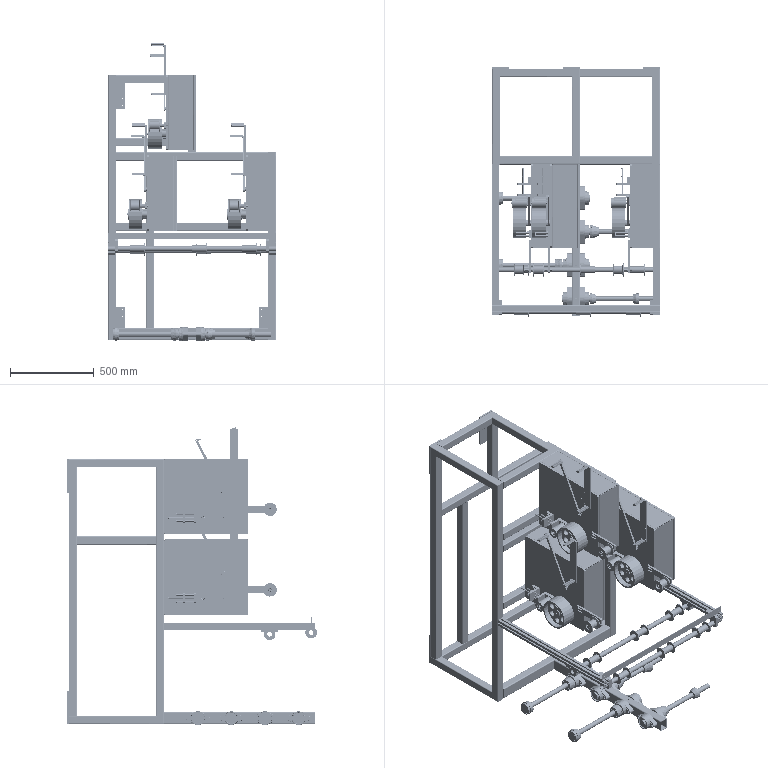Assembly | SolidWorks | mm | 185 component files | 205 solids | 13372 faces | box 1000 x 1490 x 1777.99 mm | volume 37448972 mm3 | plane 5170 | cylinder 3628 | spline 2452 | torus 1200 | sphere 624 | cone 298 | commonest cylinder face diameters 107 x315 102.497 x315 6 x255 5 x252 10 x167 4.2 x152 32.5 x120 36.5 x114
Bill of materials:
291_UCFLU206 | 8 |  | Two-bolt flange housing with a diamond/oval base. It has a raised round boss holding an inner ring with a bore, and a small protrusion on the rim that looks like a nipple.
AluminumBracket | 2 |  | Long straight bar with a square, slotted cross-section that stays the same along its length, made of four corner lobes around a central core.
Axis | 4 |  | Plain solid round rod with flat ends.
AxisSeat | 2 |  | Block with a wide flat top flange and a narrower lower body that has a large horizontal through bore and chamfered lower corners.
BearingBasePlate | 8 |  | Flat diamond-shaped plate or spacer with rounded ends, a large central hole and two small holes at the ends.
AdjustmentSeat | 3 |  | Thick L-shaped angle bracket with slotted holes in both legs and small holes in the end face of the long leg.
AngleDisplacementSensor | 3 |  | Stepped round part: a small shaft stub, a middle step and a large cylindrical head with a narrow ring groove near the shoulder.
AngleDisplacementSensorMountingPlate | 3 |  | Flat plate with two chamfered corners at the bottom, two small holes near the top and one large hole near the bottom.
AngleDisplacementSensorNut | 3 |  | Hexagonal ring shaped like a thin nut, with a large plain round bore.
AngleSensorConnectionAxis | 3 |  | Stepped round shaft with a raised collar, a hollow end with a central bore and two small cross holes near that end.
BearingHousing2 | 3 |  | Near-cubic block with a stepped (counterbored) horizontal through bore, two holes in the top face and one chamfered lower edge.
CylindricalGear35_1 | 3 | 45 | Straight-toothed spur gear with a plain central bore and radial holes through the rim into the bore.
deep groove ball bearings gb | 24 |  | Ring-shaped rolling-element assembly shape: outer ring and inner ring with a single row of spherical balls between them, resembling a radial ball bearing.
AuxiliaryWheel | 3 |  | Cylindrical sleeve with a thin raised flange at each end and a central through bore.
AuxiliaryWheelAdjustmentSeat | 3 |  | L-shaped angle bracket of roughly uniform thickness: one leg has three round holes in a line, the other leg has two parallel elongated slots.
AuxiliaryWheelFrame | 3 |  | L-shaped angle bracket: one leg has three small round holes in a line, the other leg has a single round hole.
BearingHousing | 3 |  | Thick rectangular block or plate with a large central circular through hole and four smaller round holes near the corners.
CopperSleeve10-14 | 9 |  | Plain cylindrical tube or sleeve with a concentric through bore and flat ends.
CylindricalGear105_1 | 3 | 45 | Thin flat disc-type spur gear with many small external teeth and a central bore with a single keyway notch.
ElectricalBoxCover | 3 |  | Thin flat rectangular plate or panel with no clear holes or cutouts.
GuidePlate | 3 |  | Long narrow flat bar or plate with a pattern of small round holes: two pairs of larger holes toward one end and a single smaller hole near each end.
GuidePlate2 | 3 |  | Rectangular flat bar with chamfered corners at one end, a single round hole near that end, and two parallel elongated slots near the opposite end.
GuideWheel | 3 |  | Cylindrical wheel or drum: an outer rim surrounds a recessed web with six round lightening-style holes around a central hub with a keyed bore.
M6-8-13-100GuidePinBolt | 6 |  | Headed stepped cylindrical pin: a short larger-diameter head, a long main shank, and a reduced-diameter tip section at the far end.
M6-8-13-150GuidePinBolt | 3 |  | Long, slender solid round pin. It has a short larger-diameter cylindrical head at one end and a small stepped-down end at the other.
M8-10-16-90GuidePinBolt | 3 |  | Solid round pin with a cylindrical head. The head joins a main shank through a short neck. At the far end the shank steps down through a short collar section to a reduced-diameter tip.
MotorShaftSleeve | 3 |  | Hollow cylindrical sleeve with two outside diameters. It has a keyed through-bore, and the larger-diameter section has small radial cross holes.
MotorShaftSleeve2 | 3 |  | Flanged tubular spacer: a thin circular flange at one end of a cylindrical tube with a small central through-hole.
NylonGuideBlock | 9 |  | Long rectangular-section, U-shaped fork-like bar: two parallel prongs joined at one end, leaving a long open slot between them. One prong ends in a taller block with a transverse round hole.
Part6 | 3 |  | Thin, flat rectangular plate with chamfered corners. It has two larger round holes and a pattern of many small holes.
RollerAxis | 3 |  | Round shaft with a larger cylindrical collar placed off-center along its length. The collar has a flat face on one side, and the shaft continues from both ends of the collar at slightly different diameters.
RoundNut | 3 |  | Short, thick annular ring with a large central bore and several rectangular notches spaced around its outer edge.
SmallElectricalBox | 3 |  | Thin-walled rectangular box or enclosure that is open on one large face. The opposite wall has one large round hole, one smaller round hole, and several small holes.
StepperMotor | 3 |  | Compact block-shaped body with a square end flange that has a mounting hole near each corner. A cylindrical boss projects from one end and a stepped round shaft from the other, and the body's long edges have grooves.
SwingArm | 3 |  | Long, slender rectangular-section bar or strip with a round hole near each end. The two holes appear to be different sizes.
SwingRodAxis | 3 |  | Stepped solid round shaft with several cylindrical sections, including a larger collar. It has a central hole in one end face and an elongated slot or keyway on one cylindrical section.
UpperGuideWheel | 3 |  | Axisymmetric spool/bobbin shape: cylindrical hub between two thin circular flanges whose inner faces taper toward the hub, with a central through-bore.
EndCap1 | 1 |  | Thick flat circular disc (washer-like) with a single concentric through-hole.
FootPlate | 4 |  | Thin rectangular flat plate with one larger round hole near one corner and four smaller round holes in a rectangular pattern toward the opposite end.
Frame | 1 |  | Open frame built from square/rectangular-section bar members, made up of two adjoining rectangular box frames of different heights with intermediate cross members, plus one long straight member extending outward at the base with a row of holes.
LocatingSleeve1 | 2 |  | Axisymmetric sleeve: a short cylindrical band at the large end that transitions into a truncated cone, with a large central through-bore and small radial holes in the cylindrical band.
LocatingSleeve2 | 2 |  | Axisymmetric sleeve similar to a tapered collar: a short cylindrical band at the large end followed by a longer truncated cone, a concentric through-bore, and small radial holes in the cylindrical band.
LocatingSleeve3-1 | 4 |  | Thick annular ring/flange with a large central bore, four axial through-holes on a bolt-circle-like pattern, and small radial holes through the outer cylindrical surface.
LocatingSleeve3-2 | 4 |  | Short thick cylindrical hub/disc with a large central bore and four axial through-holes in a circular pattern; side views show a slight taper of the outer surface.
Pulley | 6 |  | Spool/bobbin shape: long cylindrical hub with two thin flat circular flanges at the ends and a concentric through-bore.
StainlessSteelAxis | 2 |  | Long straight thin-walled round tube with plain square-cut ends.
SupportPlate | 1 |  | Long straight equal-leg angle (L-section) with a fillet at the inside root and rounded leg tips, and a small hole near each end of one leg.
UpperAxisBracket | 2 |  | Thick flat plate bracket with a stepped (L-like) outline and chamfered corners, a large round through-hole in the lower lobe, two smaller through-holes in the upper arm, and a small cross hole opening into the large bore.
Mates:
1. coincident | Frame-1 face at (-20.532, 1134.666, 2356.399) dir (0, 1, 0) | FootPlate-1 face at (-15.532, 1134.666, 2256.399) dir (0, -1, 0)
2. coincident | Frame-1 face at (-65.532, 1089.666, 2356.399) dir (-1, 0, 0) | FootPlate-1 face at (-65.532, 1134.666, 2156.399) dir (-1, 0, 0)
3. coincident | Frame-1 face at (-20.532, 564.666, 2356.399) dir (0, 0, 1) | FootPlate-1 face at (-65.532, 1134.666, 2356.399) dir (0, 0, 1)
4. coincident | Frame-1 face at (934.468, 1134.666, 781.399) dir (0, 1, 0) | FootPlate-2 face at (-15.532, 1134.666, 876.399) dir (0, -1, 0)
5. coincident | Frame-1 face at (-65.532, 1134.666, 781.399) dir (-1, 0, 0) | FootPlate-2 face at (-65.532, 1144.666, 976.399) dir (-1, 0, 0)
6. coincident | Frame-1 face at (-60.532, 1134.666, 776.399) dir (0, 0, -1) | FootPlate-2 face at (-65.532, 1144.666, 776.399) dir (0, 0, -1)
7. coincident | Frame-1 face at (889.468, 1134.666, 776.399) dir (0, 1, 0) | FootPlate-4 face at (884.468, 1134.666, 876.399) dir (0, -1, 0)
8. coincident | Frame-1 face at (934.468, 1089.666, 776.399) dir (1, 0, 0) | FootPlate-4 face at (934.468, 1134.666, 976.399) dir (1, 0, 0)
9. coincident | Frame-1 sketch segment at (-65.532, 564.666, 776.399) dir (0.8688, 0.4952, 0) | FootPlate-4 face at (934.468, 1134.666, 776.399) dir (0, 0, -1)
10. coincident | Frame-1 face at (459.468, 1134.666, 2311.399) dir (0, 1, 0) | FootPlate-3 face at (409.468, 1134.666, 2256.399) dir (0, -1, 0)
11. coincident | Frame-1 face at (459.468, 564.666, 2311.399) dir (1, 0, 0) | FootPlate-3 face at (459.468, 1144.666, 2156.399) dir (1, 0, 0)
12. coincident | Frame-1 face at (414.468, 564.666, 2356.399) dir (0, 0, 1) | FootPlate-3 face at (459.468, 1144.666, 2356.399) dir (0, 0, 1)
13. concentric | Frame-1 face at (-65.532, 364.666, 811.399) dir (1, 0, 0) r 17.5 | BearingBasePlate-1 face at (394.468, 364.666, 811.399) dir (1, 0, 0) r 17.5
14. coincident | Frame-1 face at (409.468, -335.334, 782.399) dir (-1, 0, 0) | BearingBasePlate-1 face at (409.468, 364.666, 811.399) dir (1, 0, 0)
15. coincident | BearingBasePlate-1 plane at (409.468, 364.666, 811.399) dir (0, 0, -1) | assembly sketch segment at (459.468, -335.334, 811.399) dir (0, 1, 0)
16. coincident | BearingBasePlate-5 face at (474.468, 364.666, 811.399) dir (1, 0, 0) | 291_UCFLU206-1 face at (474.468, 364.666, 811.399) dir (-1, 0, 0)
17. concentric | BearingBasePlate-5 face at (474.468, 306.416, 811.399) dir (1, 0, 0) r 5.1 | 291_UCFLU206-1 face at (512.468, 306.416, 811.399) dir (-1, 0, 0) r 6.5
18. concentric | BearingBasePlate-5 face at (474.468, 422.916, 811.399) dir (1, 0, 0) r 5.1 | 291_UCFLU206-1 face at (512.468, 422.916, 811.399) dir (-1, 0, 0) r 6.5
19. coincident | BearingBasePlate-6 face at (474.468, 164.666, 811.399) dir (1, 0, 0) | 291_UCFLU206-2 face at (474.468, 164.666, 811.399) dir (-1, 0, 0)
20. concentric | BearingBasePlate-6 face at (474.468, 106.416, 811.399) dir (1, 0, 0) r 5.1 | 291_UCFLU206-2 face at (512.468, 106.416, 811.399) dir (-1, 0, 0) r 6.5
21. concentric | BearingBasePlate-6 face at (474.468, 222.916, 811.399) dir (1, 0, 0) r 5.1 | 291_UCFLU206-2 face at (512.468, 222.916, 811.399) dir (-1, 0, 0) r 6.5
22. coincident | BearingBasePlate-7 face at (474.468, -35.334, 811.399) dir (1, 0, 0) | 291_UCFLU206-4 face at (474.468, -35.334, 811.399) dir (-1, 0, 0)
23. concentric | BearingBasePlate-7 face at (474.468, -93.584, 811.399) dir (1, 0, 0) r 5.1 | 291_UCFLU206-4 face at (512.468, -93.584, 811.399) dir (-1, 0, 0) r 6.5
24. concentric | BearingBasePlate-7 face at (474.468, 22.916, 811.399) dir (1, 0, 0) r 5.1 | 291_UCFLU206-4 face at (512.468, 22.916, 811.399) dir (-1, 0, 0) r 6.5
25. coincident | BearingBasePlate-8 face at (474.468, -235.334, 811.399) dir (1, 0, 0) | 291_UCFLU206-6 face at (474.468, -235.334, 811.399) dir (-1, 0, 0)
26. concentric | BearingBasePlate-8 face at (474.468, -293.584, 811.399) dir (1, 0, 0) r 5.1 | 291_UCFLU206-6 face at (512.468, -293.584, 811.399) dir (-1, 0, 0) r 6.5
27. concentric | BearingBasePlate-8 face at (474.468, -177.084, 811.399) dir (1, 0, 0) r 5.1 | 291_UCFLU206-6 face at (512.468, -177.084, 811.399) dir (-1, 0, 0) r 6.5
28. coincident | BearingBasePlate-1 face at (394.468, 364.666, 811.399) dir (-1, 0, 0) | 291_UCFLU206-8 face at (394.468, 364.666, 811.399) dir (1, 0, 0)
29. concentric | BearingBasePlate-1 face at (409.468, 306.416, 811.399) dir (1, 0, 0) r 5.1 | 291_UCFLU206-8 face at (356.468, 306.416, 811.399) dir (1, 0, 0) r 6.5
30. concentric | BearingBasePlate-1 face at (409.468, 422.916, 811.399) dir (1, 0, 0) r 5.1 | 291_UCFLU206-8 face at (356.468, 422.916, 811.399) dir (1, 0, 0) r 6.5
31. coincident | BearingBasePlate-2 face at (394.468, 164.666, 811.399) dir (-1, 0, 0) | 291_UCFLU206-10 face at (394.468, 164.666, 811.399) dir (1, 0, 0)
32. concentric | BearingBasePlate-2 face at (409.468, 106.416, 811.399) dir (1, 0, 0) r 5.1 | 291_UCFLU206-10 face at (356.468, 106.416, 811.399) dir (1, 0, 0) r 6.5
33. concentric | BearingBasePlate-2 face at (409.468, 222.916, 811.399) dir (1, 0, 0) r 5.1 | 291_UCFLU206-10 face at (356.468, 222.916, 811.399) dir (1, 0, 0) r 6.5
34. coincident | BearingBasePlate-3 face at (394.468, -35.334, 811.399) dir (-1, 0, 0) | 291_UCFLU206-12 face at (394.468, -35.334, 811.399) dir (1, 0, 0)
35. concentric | BearingBasePlate-3 face at (409.468, -93.584, 811.399) dir (1, 0, 0) r 5.1 | 291_UCFLU206-12 face at (356.468, -93.584, 811.399) dir (1, 0, 0) r 6.5
36. concentric | BearingBasePlate-3 face at (409.468, 22.916, 811.399) dir (1, 0, 0) r 5.1 | 291_UCFLU206-12 face at (356.468, 22.916, 811.399) dir (1, 0, 0) r 6.5
37. coincident | BearingBasePlate-4 face at (394.468, -235.334, 811.399) dir (-1, 0, 0) | 291_UCFLU206-14 face at (394.468, -235.334, 811.399) dir (1, 0, 0)
38. concentric | BearingBasePlate-4 face at (409.468, -293.584, 811.399) dir (1, 0, 0) r 5.1 | 291_UCFLU206-14 face at (356.468, -293.584, 811.399) dir (1, 0, 0) r 6.5
39. concentric | BearingBasePlate-4 face at (409.468, -177.084, 811.399) dir (1, 0, 0) r 5.1 | 291_UCFLU206-14 face at (356.468, -177.084, 811.399) dir (1, 0, 0) r 6.5
40. concentric | 291_UCFLU206-8 face at (394.468, 364.666, 811.399) dir (1, 0, 0) r 15 | Axis-4 face at (516.668, 364.666, 811.399) dir (-1, 0, 0) r 15
41. coincident | 291_UCFLU206-1 face at (516.668, 379.515, 796.549) dir (1, 0, 0) | Axis-4 face at (516.668, 364.666, 811.399) dir (1, 0, 0)
42. concentric | 291_UCFLU206-2 face at (474.468, 164.666, 811.399) dir (-1, 0, 0) r 15 | Axis-1 face at (352.268, 164.666, 811.399) dir (1, 0, 0) r 15
43. concentric | 291_UCFLU206-4 face at (474.468, -35.334, 811.399) dir (-1, 0, 0) r 15 | Axis-2 face at (-38.332, -35.334, 811.399) dir (1, 0, 0) r 15
44. concentric | 291_UCFLU206-6 face at (474.468, -235.334, 811.399) dir (-1, 0, 0) r 15 | Axis-3 face at (352.268, -235.334, 811.399) dir (1, 0, 0) r 15
45. coincident | 291_UCFLU206-4 face at (516.668, -20.485, 796.549) dir (1, 0, 0) | Axis-2 face at (516.668, -35.334, 811.399) dir (1, 0, 0)
46. coincident | 291_UCFLU206-14 face at (352.268, -220.485, 826.248) dir (-1, 0, 0) | Axis-3 face at (352.268, -235.334, 811.399) dir (-1, 0, 0)
47. coincident | 291_UCFLU206-10 face at (352.268, 179.515, 826.248) dir (-1, 0, 0) | Axis-1 face at (352.268, 164.666, 811.399) dir (-1, 0, 0)
48. coincident | Frame-1 face at (-20.532, 564.666, 776.399) dir (0, -1, 0) | AluminumBracket-2 face at (-26.032, 564.666, 1375.899) dir (0, 1, 0)
49. coincident | Frame-1 face at (889.468, 564.666, 1896.399) dir (0, -1, 0) | AluminumBracket-1 face at (933.968, 564.666, 1375.899) dir (0, 1, 0)
50. coincident | Frame-1 face at (934.468, 609.666, 1896.399) dir (1, 0, 0) | AluminumBracket-1 face at (934.468, 564.666, 1360.399) dir (1, 0, 0)
51. coincident | Frame-1 face at (-65.532, 609.666, 776.399) dir (-1, 0, 0) | AluminumBracket-2 face at (-65.532, 564.666, 1336.899) dir (-1, 0, 0)
52. distance | AluminumBracket-2 face at (-49.532, 564.666, 1336.399) dir (0, 0, -1) | Frame-1 face at (-60.532, 1134.666, 776.399) dir (0, 0, -1)
53. distance | AluminumBracket-1 face at (933.968, 564.666, 1336.399) dir (0, 0, -1) | Frame-1 face at (889.468, 564.666, 776.399) dir (0, 0, -1)
54. coincident | AluminumBracket-1 face at (933.968, 564.666, 1336.399) dir (0, 0, -1) | AxisSeat-1 face at (894.468, -112.684, 1336.399) dir (0, 0, 1)
55. coincident | AluminumBracket-1 face at (934.468, 564.666, 1336.899) dir (1, 0, 0) | AxisSeat-1 face at (934.468, -62.684, 1336.399) dir (1, 0, 0)
56. coincident | AluminumBracket-2 face at (-26.032, 564.666, 1336.399) dir (0, 0, -1) | AxisSeat-2 face at (-65.532, -112.684, 1336.399) dir (0, 0, 1)
57. coincident | AluminumBracket-2 face at (-65.532, 564.666, 1336.899) dir (-1, 0, 0) | AxisSeat-2 face at (-65.532, -62.684, 1336.399) dir (-1, 0, 0)
58. concentric | AxisSeat-1 face at (894.468, -62.684, 1311.399) dir (1, 0, 0) r 15 | StainlessSteelAxis-2 face at (-65.532, -62.684, 1311.399) dir (1, 0, 0) r 15
59. lock | AluminumBracket-1 reference at (0, 0, 0) dir (1, 0, 0) | AxisSeat-1 reference at (0, 0, 0) dir (1, 0, 0)
60. coincident | AxisSeat-2 face at (-65.532, -62.684, 1336.399) dir (-1, 0, 0) | StainlessSteelAxis-2 edge at (-65.532, -62.684, 1311.399) dir (-1, 0, 0) r 14
61. coincident | AluminumBracket-1 face at (894.468, 564.666, 1336.899) dir (-1, 0, 0) | UpperAxisBracket-2 face at (894.468, -245.334, 1376.399) dir (1, 0, 0)
62. coincident | AluminumBracket-1 face at (910.468, 564.666, 1376.399) dir (0, 0, 1) | UpperAxisBracket-2 face at (874.468, -245.334, 1376.399) dir (0, 0, 1)
63. coincident | AluminumBracket-2 face at (-25.532, 564.666, 1360.399) dir (1, 0, 0) | UpperAxisBracket-1 face at (-25.532, -245.334, 1376.399) dir (-1, 0, 0)
64. coincident | AluminumBracket-2 edge at (-26.032, 564.666, 1376.399) dir (0, -1, 0) | UpperAxisBracket-1 face at (-25.532, -245.334, 1376.399) dir (0, 0, 1)
65. coincident | AluminumBracket-2 face at (-26.032, -335.334, 1375.899) dir (0, -1, 0) | UpperAxisBracket-1 face at (-25.532, -335.334, 1376.399) dir (0, -1, 0)
66. coincident | AluminumBracket-1 face at (933.968, -335.334, 1375.899) dir (0, -1, 0) | UpperAxisBracket-2 face at (874.468, -335.334, 1376.399) dir (0, -1, 0)
67. concentric | StainlessSteelAxis-1 face at (-65.532, -310.334, 1321.399) dir (1, 0, 0) r 15 | UpperAxisBracket-2 face at (874.468, -310.334, 1321.399) dir (1, 0, 0) r 15
68. coincident | AluminumBracket-2 face at (-65.532, 564.666, 1336.899) dir (-1, 0, 0) | StainlessSteelAxis-1 face at (-65.532, -310.334, 1321.399) dir (-1, 0, 0)
69. concentric | StainlessSteelAxis-2 face at (-65.532, -62.684, 1311.399) dir (1, 0, 0) r 15 | Pulley-6 face at (62.13, -62.684, 1311.399) dir (-1, 0, 0) r 15
70. concentric | StainlessSteelAxis-2 face at (-65.532, -62.684, 1311.399) dir (1, 0, 0) r 15 | Pulley-5 face at (754.182, -62.684, 1311.399) dir (-1, 0, 0) r 15
71. concentric | StainlessSteelAxis-2 face at (-65.532, -62.684, 1311.399) dir (1, 0, 0) r 15 | Pulley-4 face at (459.502, -62.684, 1311.399) dir (-1, 0, 0) r 15
72. concentric | StainlessSteelAxis-1 face at (-65.532, -310.334, 1321.399) dir (1, 0, 0) r 15 | Pulley-3 face at (62.354, -310.334, 1321.399) dir (-1, 0, 0) r 15
73. concentric | StainlessSteelAxis-1 face at (-65.532, -310.334, 1321.399) dir (1, 0, 0) r 15 | Pulley-2 face at (433.04, -310.334, 1321.399) dir (-1, 0, 0) r 15
74. concentric | StainlessSteelAxis-1 face at (-65.532, -310.334, 1321.399) dir (1, 0, 0) r 15 | Pulley-1 face at (730.2, -310.334, 1321.399) dir (-1, 0, 0) r 15
75. concentric | Axis-2 face at (-38.332, -35.334, 811.399) dir (1, 0, 0) r 15 | LocatingSleeve3-1/LocatingSleeve3-1-1 face at (352.268, -35.334, 811.399) dir (1, 0, 0) r 15
76. coincident | 291_UCFLU206-12 face at (352.268, -20.485, 826.248) dir (-1, 0, 0) | LocatingSleeve3-1/LocatingSleeve3-1-1 face at (352.268, -27.137, 798.837) dir (1, 0, 0)
77. concentric | Axis-4 face at (516.668, 364.666, 811.399) dir (-1, 0, 0) r 15 | LocatingSleeve3-2/LocatingSleeve3-2-1 face at (338.268, 364.666, 811.399) dir (1, 0, 0) r 15
78. coincident | 291_UCFLU206-8 face at (352.268, 379.515, 826.248) dir (-1, 0, 0) | LocatingSleeve3-2/LocatingSleeve3-1-1 face at (352.268, 373.123, 799.01) dir (1, 0, 0)
79. concentric | Axis-4 face at (516.668, 364.666, 811.399) dir (-1, 0, 0) r 15 | LocatingSleeve3-3/LocatingSleeve3-1-1 face at (-38.332, 364.666, 811.399) dir (-1, 0, 0) r 15
80. coincident | Axis-2 face at (-38.332, -35.334, 811.399) dir (1, 0, 0) r 15 | LocatingSleeve3-4/LocatingSleeve3-1-1 edge at (-24.332, -35.334, 811.399) dir (-1, 0, 0) r 15
81. coincident | Axis-2 face at (-38.332, -35.334, 811.399) dir (-1, 0, 0) | LocatingSleeve3-4/LocatingSleeve3-1-1 face at (-38.332, -24.324, 821.586) dir (-1, 0, 0)
82. coincident | Axis-4 face at (-38.332, 364.666, 811.399) dir (-1, 0, 0) | LocatingSleeve3-3/LocatingSleeve3-1-1 face at (-38.332, 372.22, 824.358) dir (-1, 0, 0)
83. concentric | Axis-3 face at (352.268, -235.334, 811.399) dir (1, 0, 0) r 15 | LocatingSleeve1-1 face at (516.668, -235.334, 811.399) dir (-1, 0, 0) r 15
84. coincident | 291_UCFLU206-6 face at (516.668, -220.485, 796.549) dir (1, 0, 0) | LocatingSleeve1-1 face at (516.668, -221.244, 806.254) dir (-1, 0, 0)
85. concentric | Axis-3 face at (352.268, -235.334, 811.399) dir (1, 0, 0) r 15 | LocatingSleeve1-2 face at (807.268, -235.334, 811.399) dir (1, 0, 0) r 15
86. distance | LocatingSleeve1-2 face at (807.268, -220.694, 814.666) dir (1, 0, 0) | Axis-3 face at (907.268, -235.334, 811.399) dir (1, 0, 0)
87. concentric | Axis-1 face at (352.268, 164.666, 811.399) dir (1, 0, 0) r 15 | LocatingSleeve2-1 face at (516.668, 164.666, 811.399) dir (-1, 0, 0) r 15
88. coincident | 291_UCFLU206-2 face at (516.668, 179.515, 796.549) dir (1, 0, 0) | LocatingSleeve2-1 face at (516.668, 154.643, 800.239) dir (-1, 0, 0)
89. concentric | Axis-1 face at (352.268, 164.666, 811.399) dir (1, 0, 0) r 15 | LocatingSleeve2-2 face at (807.268, 164.666, 811.399) dir (1, 0, 0) r 15
90. distance | LocatingSleeve2-2 face at (807.268, 163.044, 826.311) dir (1, 0, 0) | Axis-1 face at (907.268, 164.666, 811.399) dir (1, 0, 0)
91. coincident | AxisSeat-1 face at (894.468, -92.684, 1286.399) dir (0, -1, 0) | AxisSeat-2 face at (-65.532, -92.684, 1286.399) dir (0, -1, 0)
92. coincident | Frame-1 face at (-65.532, 564.666, 1851.399) dir (0, -1, 0) | ElectricalBoxAssembly2-1/Part6-1 face at (755.468, 564.666, 1876.399) dir (0, 1, 0)
93. distance | ElectricalBoxAssembly2-1/Part6-1 face at (767.468, 314.666, 1651.399) dir (1, 0, 0) | Frame-1 face at (934.468, 609.666, 1896.399) dir (1, 0, 0)
94. coincident | Frame-1 face at (-20.532, 564.666, 776.399) dir (0, -1, 0) | ElectricalBoxAssembly2-2/Part6-1 face at (164.468, 564.666, 1876.399) dir (0, 1, 0)
95. distance | ElectricalBoxAssembly2-2/Part6-1 face at (164.468, 314.666, 1651.399) dir (-1, 0, 0) | Frame-1 face at (-65.532, 609.666, 776.399) dir (-1, 0, 0)
96. coincident | Frame-1 face at (-65.532, 564.666, 2311.399) dir (0, -1, 0) | ElectricalBoxAssembly2-3/Part6-1 face at (280.468, 564.666, 2356.399) dir (0, 1, 0)
97. coincident | Frame-1 face at (-65.532, 609.666, 2356.399) dir (0, 0, 1) | ElectricalBoxAssembly2-3/Part6-1 face at (280.468, 64.666, 2356.399) dir (0, 0, 1)
98. distance | ElectricalBoxAssembly2-3/Part6-1 face at (292.468, 314.666, 2131.399) dir (1, 0, 0) | Frame-1 face at (459.468, 564.666, 2311.399) dir (1, 0, 0)
99. coincident | Frame-1 face at (-65.532, 569.666, 1426.399) dir (0, 0, -1) | ElectricalBoxAssembly2-1/Part6-1 face at (755.468, 64.666, 1426.399) dir (0, 0, -1)
100. coincident | Frame-1 face at (-65.532, 569.666, 1426.399) dir (0, 0, -1) | ElectricalBoxAssembly2-2/Part6-1 face at (164.468, 64.666, 1426.399) dir (0, 0, -1)
101. coincident | AluminumBracket-1 face at (910.468, 564.666, 1376.399) dir (0, 0, 1) | SupportPlate-1 face at (934.468, -275.334, 1376.399) dir (0, 0, -1)
102. coincident | AluminumBracket-1 face at (934.468, 564.666, 1360.399) dir (1, 0, 0) | SupportPlate-1 face at (934.468, -313.334, 1415.399) dir (1, 0, 0)
103. distance | SupportPlate-1 face at (934.468, -315.334, 1376.399) dir (0, -1, 0) | AluminumBracket-1 face at (933.968, -335.334, 1375.899) dir (0, -1, 0)
104. coincident | ElectricalBoxAssembly2-3/deep groove ball bearings gb-2 face at (181.468, -73.001, 2056.399) dir (-1, 0, 0) | EndCap1-1 face at (181.468, -65.334, 2056.399) dir (1, 0, 0)
105. concentric | ElectricalBoxAssembly2-3/RollerAxis-1 face at (178.468, -65.334, 2056.399) dir (-1, 0, 0) r 2.5 | EndCap1-1 face at (176.468, -65.334, 2056.399) dir (-1, 0, 0) r 3.3
106. coincident | Part6-1 plane at (-18.103, -45.257, 494) dir (1, 0, 0) | SmallElectricalBox-1 plane at (-18.103, -45.257, 344) dir (-1, 0, 0)
107. coincident | Part6-1 plane at (-18.103, -45.257, 494) dir (0, 1, 0) | SmallElectricalBox-1 plane at (-18.103, -45.257, 344) dir (0, -1, 0)
108. coincident | Part6-1 face at (-18.103, -45.257, 494) dir (0, 0, -1) | SmallElectricalBox-1 face at (-18.103, -45.257, 494) dir (0, 0, 1)
109. concentric | Part6-1 face at (106.897, 54.743, 506) dir (0, 0, -1) r 22.5 | StepperMotor-1 face at (106.897, 54.743, 533.5) dir (0, 0, -1) r 9.5
110. parallel | Part6-1 face at (206.897, 204.743, 506) dir (1, 0, 0) | StepperMotor-1 face at (161.897, 109.743, 492.5) dir (1, 0, 0)
111. coincident | SmallElectricalBox-1 face at (-18.103, -45.257, 492.5) dir (0, 0, -1) | StepperMotor-1 face at (106.897, 54.743, 492.5) dir (0, 0, 1)
112. concentric | StepperMotor-1 face at (106.897, 54.743, 533.5) dir (0, 0, -1) r 9.5 | MotorShaftSleeve-1 face at (106.897, 54.743, 582.5) dir (0, 0, -1) r 9.5
113. parallel | StepperMotor-1 face at (106.897, 61.243, 553.5) dir (0, 1, 0) | MotorShaftSleeve-1 face at (109.897, 66.756, 582.5) dir (0, -1, 0)
114. coincident | StepperMotor-1 face at (106.897, 54.743, 499.5) dir (0, 0, 1) | MotorShaftSleeve-1 face at (106.897, 54.743, 499.5) dir (0, 0, -1)
115. concentric | MotorShaftSleeve-1 face at (106.897, 54.743, 582.5) dir (0, 0, -1) r 17.5 | GuideWheel-1 face at (106.897, 54.743, 613) dir (0, 0, -1) r 17.5
116. parallel | MotorShaftSleeve-1 face at (106.897, 41.243, 572.5) dir (0, -1, 0) | GuideWheel-1 face at (102.897, 34.079, 533) dir (0, 1, 0)
117. concentric | MotorShaftSleeve-1 face at (106.897, 54.743, 582.5) dir (0, 0, -1) r 9.5 | MotorShaftSleeve2-1 face at (106.897, 54.743, 538) dir (0, 0, 1) r 9.5
118. concentric | Part6-1 edge at (-223.103, 138.131, 506) dir (0, 0, 1) r 2.1 | GuidePlate-1 face at (-223.103, 138.131, 506) dir (0, 0, 1) r 3
119. concentric | Part6-1 face at (-143.103, 138.131, 506) dir (0, 0, 1) r 2.1 | GuidePlate-1 face at (-143.103, 138.131, 506) dir (0, 0, 1) r 3
120. coincident | Part6-1 face at (-18.103, -45.257, 506) dir (0, 0, 1) | GuidePlate-1 face at (-273.103, 119.743, 506) dir (0, 0, -1)
121. coincident | Part6-1 face at (-18.103, -45.257, 506) dir (0, 0, 1) | GuidePlate2-1 face at (56.897, 254.743, 506) dir (0, 0, -1)
122. distance | GuidePlate2-1 face at (76.897, 354.743, 518) dir (1, 0, 0) | Part6-1 face at (206.897, 204.743, 506) dir (1, 0, 0)
123. distance | GuidePlate2-1 face at (76.897, 154.743, 518) dir (0, -1, 0) | Part6-1 face at (-243.103, 204.743, 506) dir (0, 1, 0)
124. concentric | Part6-1 face at (-43.103, 54.743, 506) dir (0, 0, -1) r 10 | SwingArm-1 face at (-43.103, 54.743, 521) dir (0, 0, -1) r 5
125. concentric | GuidePlate2-1 face at (56.897, 334.743, 518) dir (0, 0, 1) r 4 | RollerAxis-1 face at (56.897, 334.743, 496) dir (0, 0, -1) r 4
126. coincident | GuidePlate2-1 face at (56.897, 254.743, 518) dir (0, 0, 1) | RollerAxis-1 face at (53.907, 337.4, 518) dir (0, 0, -1)
127. concentric | RollerAxis-1 face at (56.897, 334.743, 496) dir (0, 0, -1) r 5 | UpperGuideWheel-1 face at (56.897, 334.743, 533.465) dir (0, 0, -1) r 12.5
128. coincident | RollerAxis-1 face at (49.422, 341.385, 543) dir (0, 0, 1) | UpperGuideWheel-1 face at (58.388, 352.179, 543) dir (0, 0, -1)
129. concentric | RollerAxis-1 face at (56.897, 334.743, 496) dir (0, 0, -1) r 5 | deep groove ball bearings gb-1 face at (56.897, 334.743, 543.029) dir (0, 0, -1) r 5
130. coincident | UpperGuideWheel-1 face at (58.388, 352.179, 554) dir (0, 0, -1) | deep groove ball bearings gb-1 face at (58.544, 347.638, 554) dir (0, 0, 1)
131. concentric | RollerAxis-1 face at (56.897, 334.743, 496) dir (0, 0, -1) r 5 | deep groove ball bearings gb-2 face at (56.897, 334.743, 607.971) dir (0, 0, 1) r 5
132. coincident | UpperGuideWheel-1 face at (57.962, 347.197, 597) dir (0, 0, 1) | deep groove ball bearings gb-2 face at (56.897, 347.743, 597) dir (0, 0, -1)
133. coincident | SmallElectricalBox-1 face at (-243.103, -295.257, 494) dir (-1, 0, 0) | ElectricalBoxCover-1 face at (-243.103, -45.257, 329) dir (-1, 0, 0)
134. coincident | SmallElectricalBox-1 face at (206.897, 204.743, 494) dir (0, 1, 0) | ElectricalBoxCover-1 face at (-18.103, 204.743, 329) dir (0, 1, 0)
135. coincident | SmallElectricalBox-1 face at (-18.103, -45.257, 344) dir (0, 0, -1) | ElectricalBoxCover-1 face at (-18.103, -45.257, 344) dir (0, 0, 1)
136. coincident | Part6-1 face at (-18.103, -45.257, 506) dir (0, 0, 1) | AuxiliaryWheelAdjustmentSeat-1 face at (136.897, -220.257, 506) dir (0, 0, -1)
137. distance | AuxiliaryWheelAdjustmentSeat-1 plane at (106.897, -220.257, 506) dir (1, 0, 0) | Part6-1 face at (206.897, 204.743, 506) dir (1, 0, 0)
138. distance | AuxiliaryWheelAdjustmentSeat-1 face at (136.897, -220.257, 521) dir (0, -1, 0) | Part6-1 face at (-243.103, -295.257, 506) dir (0, -1, 0)
139. coincident | Part6-1 face at (-18.103, -45.257, 506) dir (0, 0, 1) | AuxiliaryWheelFrame-1 face at (76.897, -120.257, 506) dir (0, 0, -1)
140. distance | AuxiliaryWheelFrame-1 plane at (106.897, -120.257, 506) dir (-1, 0, 0) | Part6-1 face at (206.897, 204.743, 506) dir (1, 0, 0)
141. concentric | SwingArm-1 face at (-354.676, -104.701, 521) dir (0, 0, 1) r 2.1 | NylonGuideBlock-1 face at (-354.676, -104.701, 601) dir (0, 0, -1) r 3
142. coincident | SwingArm-1 face at (-194.438, -22.702, 521) dir (0, 0, 1) | NylonGuideBlock-1 face at (-361.921, -93.354, 521) dir (0, 0, -1)
143. concentric | GuidePlate-1 face at (-418.103, 107.243, 506) dir (0, 0, -1) r 2.1 | NylonGuideBlock-2 face at (-418.103, 107.243, 596) dir (0, 0, -1) r 3
144. coincident | GuidePlate-1 face at (-273.103, 119.743, 516) dir (0, 0, 1) | NylonGuideBlock-2 face at (-427.65, 116.735, 516) dir (0, 0, -1)
145. concentric | GuidePlate-1 face at (-128.103, 107.243, 506) dir (0, 0, -1) r 2.1 | NylonGuideBlock-3 face at (-128.103, 107.243, 596) dir (0, 0, -1) r 3
146. coincident | GuidePlate-1 face at (-273.103, 119.743, 516) dir (0, 0, 1) | NylonGuideBlock-3 face at (-135.161, 118.707, 516) dir (0, 0, -1)
147. concentric | AuxiliaryWheel-1 face at (106.897, -65.257, 631.75) dir (0, 0, 1) r 14 | AuxiliaryWheelFrame-1 face at (106.897, -65.257, 526) dir (0, 0, 1) r 4
148. distance | Part6-1 face at (-18.103, -45.257, 506) dir (0, 0, 1) | AuxiliaryWheel-1 face at (94.781, -95.414, 530.5) dir (0, 0, -1)
149. tangent | GuideWheel-1 face at (106.897, 54.743, 613) dir (0, 0, -1) r 90 | AuxiliaryWheel-1 face at (106.897, -65.257, 631.75) dir (0, 0, 1) r 30
150. concentric | AuxiliaryWheel-1 face at (106.897, -65.257, 631.75) dir (0, 0, 1) r 17.5 | deep groove ball bearings gb-4 face at (106.897, -65.257, 617.211) dir (0, 0, 1) r 13
151. coincident | AuxiliaryWheel-1 face at (100.373, -81.496, 604.5) dir (0, 0, 1) | deep groove ball bearings gb-4 face at (106.897, -52.257, 604.5) dir (0, 0, -1)
152. concentric | AuxiliaryWheel-1 face at (106.897, -65.257, 631.75) dir (0, 0, 1) r 17.5 | deep groove ball bearings gb-3 face at (106.897, -65.257, 546.211) dir (0, 0, 1) r 13
153. coincident | AuxiliaryWheel-1 face at (100.373, -81.496, 541.5) dir (0, 0, -1) | deep groove ball bearings gb-3 face at (106.897, -52.257, 541.5) dir (0, 0, 1)
154. distance | GuideWheel-1 face at (106.897, 54.743, 533) dir (0, 0, -1) | Part6-1 face at (-18.103, -45.257, 506) dir (0, 0, 1)
155. coincident | GuideWheel-1 face at (106.897, 54.743, 583) dir (0, 0, 1) | MotorShaftSleeve2-1 face at (106.897, 54.743, 583) dir (0, 0, -1)
156. coincident | SmallElectricalBox-1 face at (-18.103, -45.257, 492.5) dir (0, 0, -1) | BearingHousing-1 face at (-43.103, 54.743, 492.5) dir (0, 0, 1)
157. concentric | Part6-1 face at (-43.103, 54.743, 506) dir (0, 0, -1) r 10 | BearingHousing-1 face at (-43.103, 54.743, 477.5) dir (0, 0, 1) r 11
158. parallel | SmallElectricalBox-1 face at (206.897, 203.243, 494) dir (0, -1, 0) | BearingHousing-1 face at (-73.103, 74.743, 492.5) dir (0, 1, 0)
159. concentric | BearingHousing-1 face at (-43.103, 54.743, 484.5) dir (0, 0, 1) r 14 | deep groove ball bearings gb-6 face at (-43.103, 54.743, 479.789) dir (0, 0, -1) r 13
160. coincident | BearingHousing-1 face at (-43.103, 54.743, 484.5) dir (0, 0, 1) | deep groove ball bearings gb-6 face at (-45.239, 67.566, 484.5) dir (0, 0, -1)
161. distance | SwingArm-1 face at (-194.438, -22.702, 511) dir (0, 0, -1) | Part6-1 face at (-18.103, -45.257, 506) dir (0, 0, 1)
162. concentric | deep groove ball bearings gb-6 face at (-43.103, 54.743, 481.529) dir (0, 0, -1) r 5 | SwingRodAxis-1 face at (-43.103, 54.743, 484.5) dir (0, 0, -1) r 10
163. coincident | deep groove ball bearings gb-6 face at (-44.363, 62.305, 484.5) dir (0, 0, -1) | SwingRodAxis-1 face at (-43.103, 54.743, 484.5) dir (0, 0, 1)
164. concentric | Part6-1 face at (-43.103, 54.743, 496) dir (0, 0, 1) r 14 | deep groove ball bearings gb-8 face at (-43.103, 54.743, 491.289) dir (0, 0, -1) r 13
165. coincident | Part6-1 face at (-43.103, 54.743, 496) dir (0, 0, 1) | deep groove ball bearings gb-8 face at (-44.242, 67.693, 496) dir (0, 0, -1)
166. concentric | SwingRodAxis-1 face at (-43.103, 54.743, 511) dir (0, 0, -1) r 6 | RoundNut-1 face at (-43.103, 54.743, 510) dir (0, 0, -1) r 6
167. coincident | deep groove ball bearings gb-8 face at (-43.541, 59.723, 504) dir (0, 0, 1) | RoundNut-1 face at (-43.103, 54.743, 504) dir (0, 0, -1)
168. concentric | SwingRodAxis-1 face at (-43.103, 54.743, 464.5) dir (0, 0, 1) r 8 | CylindricalGear105_1-1 face at (-43.103, 54.743, 474.5) dir (0, 0, -1) r 8
169. coincident | SwingRodAxis-1 face at (-43.103, 54.743, 474.5) dir (0, 0, -1) | CylindricalGear105_1-1 face at (-43.103, 54.743, 474.5) dir (0, 0, 1)
170. parallel | SwingRodAxis-1 face at (-37.762, 57.476, 471.5) dir (0.8902, 0.4556, 0) | CylindricalGear105_1-1 face at (-33.29, 57.518, 474.5) dir (-0.8902, -0.4556, 0)
171. coincident | SwingArm-1 plane at (-194.438, -22.702, 511) dir (-0.4556, 0.8902, 0) | SwingRodAxis-1 plane at (-43.103, 54.743, 474.5) dir (-0.4556, 0.8902, 0)
172. distance | AngleSensorComponentAssembly3-1/AdjustmentSeat-1 face at (-133.103, 72.243, 492.353) dir (0, 1, 0) | SmallElectricalBox-1 face at (206.897, 204.743, 494) dir (0, 1, 0)
173. distance | AngleSensorComponentAssembly3-1/AdjustmentSeat-1 face at (-173.103, 37.243, 482.353) dir (-1, 0, 0) | SmallElectricalBox-1 face at (-243.103, -295.257, 494) dir (-1, 0, 0)
174. concentric | deep groove ball bearings gb-4 face at (106.897, -65.257, 615.471) dir (0, 0, 1) r 5 | M8-10-16-90GuidePinBolt-1 face at (106.897, -65.257, 525.5) dir (0, 0, 1) r 5
175. coincident | AuxiliaryWheel-1 face at (100.373, -81.496, 615.5) dir (0, 0, 1) | M8-10-16-90GuidePinBolt-1 face at (106.897, -65.257, 615.5) dir (0, 0, -1)
176. concentric | AuxiliaryWheelFrame-1 face at (126.897, -105.257, 551) dir (0, 1, 0) r 3 | M6-8-13-100GuidePinBolt-1 face at (126.897, -110.257, 551) dir (0, -1, 0) r 3
177. coincident | AuxiliaryWheelFrame-1 face at (76.897, -120.257, 586) dir (0, -1, 0) | M6-8-13-100GuidePinBolt-1 face at (126.897, -120.257, 551) dir (0, 1, 0)
178. concentric | AuxiliaryWheelFrame-1 face at (86.897, -105.257, 551) dir (0, 1, 0) r 3 | M6-8-13-100GuidePinBolt-2 face at (86.897, -110.257, 551) dir (0, -1, 0) r 3
179. coincident | AuxiliaryWheelFrame-1 face at (76.897, -120.257, 586) dir (0, -1, 0) | M6-8-13-100GuidePinBolt-2 face at (86.897, -120.257, 551) dir (0, 1, 0)
180. concentric | AuxiliaryWheelAdjustmentSeat-1 face at (126.897, -170.257, 551) dir (0, -1, 0) r 6 | CopperSleeve10-14-1 face at (126.897, -170.257, 551) dir (0, -1, 0) r 6
181. coincident | AuxiliaryWheelAdjustmentSeat-1 face at (136.897, -170.257, 506) dir (0, 1, 0) | CopperSleeve10-14-1 face at (126.897, -170.257, 551) dir (0, 1, 0)
182. concentric | AuxiliaryWheelAdjustmentSeat-1 face at (86.897, -170.257, 551) dir (0, -1, 0) r 6 | CopperSleeve10-14-2 face at (86.897, -170.257, 551) dir (0, -1, 0) r 6
183. coincident | AuxiliaryWheelAdjustmentSeat-1 face at (136.897, -170.257, 506) dir (0, 1, 0) | CopperSleeve10-14-2 face at (86.897, -170.257, 551) dir (0, 1, 0)
184. concentric | AuxiliaryWheelAdjustmentSeat-1 face at (106.897, -170.257, 551) dir (0, -1, 0) r 6 | CopperSleeve10-14-3 face at (106.897, -170.257, 551) dir (0, -1, 0) r 6
185. coincident | AuxiliaryWheelAdjustmentSeat-1 face at (136.897, -170.257, 506) dir (0, 1, 0) | CopperSleeve10-14-3 face at (106.897, -170.257, 551) dir (0, 1, 0)
186. concentric | AuxiliaryWheelFrame-1 face at (106.897, -105.257, 551) dir (0, 1, 0) r 3 | M6-8-13-150GuidePinBolt-1 face at (106.897, -120.257, 551) dir (0, -1, 0) r 4
187. coincident | AuxiliaryWheelFrame-1 face at (76.897, -120.257, 586) dir (0, -1, 0) | M6-8-13-150GuidePinBolt-1 face at (106.897, -120.257, 551) dir (0, 1, 0)
188. coincident | AdjustmentSeat-1 plane at (-21.133, -35.026, 80) dir (0, 0, 1) | BearingHousing2-1 plane at (-41.133, 19.974, 80) dir (0, 0, 1)
189. coincident | AdjustmentSeat-1 face at (-21.133, -35.026, 97.5) dir (-1, 0, 0) | BearingHousing2-1 face at (-21.133, 4.974, 97.5) dir (1, 0, 0)
190. concentric | BearingHousing2-1 face at (-41.133, 26.974, 80) dir (0, 1, 0) r 14 | deep groove ball bearings gb-2 face at (-41.133, 39.684, 80) dir (0, 1, 0) r 13
191. coincident | BearingHousing2-1 face at (-41.133, 26.974, 80) dir (0, 1, 0) | deep groove ball bearings gb-2 face at (-29.58, 26.974, 85.961) dir (0, -1, 0)
192. concentric | BearingHousing2-1 face at (-41.133, 12.974, 80) dir (0, -1, 0) r 14 | deep groove ball bearings gb-3 face at (-41.133, 17.684, 80) dir (0, 1, 0) r 13
193. coincident | BearingHousing2-1 face at (-41.133, 12.974, 80) dir (0, -1, 0) | deep groove ball bearings gb-3 face at (-28.133, 12.974, 80) dir (0, 1, 0)
194. distance | CylindricalGear35_1-1 face at (-41.133, -7.026, 80) dir (0, 1, 0) | BearingHousing2-1 face at (-41.133, 4.974, 80) dir (0, -1, 0)
195. distance | BearingHousing2-1 face at (-41.133, 4.974, 80) dir (0, -1, 0) | AdjustmentSeat-1 face at (18.867, -35.026, 97.5) dir (0, -1, 0)
196. concentric | BearingHousing2-1 face at (-41.133, 34.974, 80) dir (0, -1, 0) r 7.5 | AngleSensorConnectionAxis-1 face at (-41.133, 44.974, 80) dir (0, -1, 0) r 6
197. coincident | BearingHousing2-1 face at (-41.133, 4.974, 80) dir (0, -1, 0) | AngleSensorConnectionAxis-1 face at (-41.133, 4.974, 80) dir (0, 1, 0)
198. concentric | CylindricalGear35_1-1 face at (-41.133, -7.026, 80) dir (0, -1, 0) r 6 | AngleSensorConnectionAxis-1 face at (-41.133, -7.026, 80) dir (0, -1, 0) r 6
199. concentric | AdjustmentSeat-1 face at (-16.133, 54.974, 70) dir (0, 1, 0) r 2.1 | AngleDisplacementSensorMountingPlate-1 face at (-16.133, 57.974, 70) dir (0, -1, 0) r 2.75
200. concentric | AdjustmentSeat-1 face at (-16.133, 54.974, 90) dir (0, 1, 0) r 2.1 | AngleDisplacementSensorMountingPlate-1 face at (-16.133, 57.974, 90) dir (0, -1, 0) r 2.75
201. coincident | AdjustmentSeat-1 face at (-21.133, 54.974, 97.5) dir (0, 1, 0) | AngleDisplacementSensorMountingPlate-1 face at (-31.133, 54.974, 80) dir (0, -1, 0)
202. concentric | AngleDisplacementSensorMountingPlate-1 face at (-41.133, 57.974, 80) dir (0, -1, 0) r 6 | AngleDisplacementSensor-1 face at (-41.133, 56.974, 80) dir (0, 1, 0) r 6
203. coincident | AngleDisplacementSensorMountingPlate-1 face at (-31.133, 57.974, 80) dir (0, 1, 0) | AngleDisplacementSensor-1 face at (-41.133, 57.974, 80) dir (0, -1, 0)
204. concentric | AngleDisplacementSensor-1 face at (-41.133, 49.974, 80) dir (0, 1, 0) r 5 | AngleDisplacementSensorNut-1 face at (-41.133, 51.974, 80) dir (0, -1, 0) r 5
205. coincident | AngleDisplacementSensorMountingPlate-1 face at (-31.133, 54.974, 80) dir (0, -1, 0) | AngleDisplacementSensorNut-1 face at (-41.133, 54.974, 80) dir (0, 1, 0)
206. concentric | LocatingSleeve3-1-1 face at (15.278, 33.35, 57.924) dir (-1, 0, 0) r 15 | LocatingSleeve3-2-1 face at (29.278, 33.35, 57.924) dir (-1, 0, 0) r 15
207. coincident | LocatingSleeve3-1-1 face at (29.278, 68.35, 57.924) dir (1, 0, 0) | LocatingSleeve3-2-1 face at (29.278, 48.35, 57.924) dir (-1, 0, 0)
208. concentric | LocatingSleeve3-1-1 face at (29.278, 60.85, 57.924) dir (1, 0, 0) r 2.5 | LocatingSleeve3-2-1 face at (55.278, 60.85, 57.924) dir (1, 0, 0) r 3.3